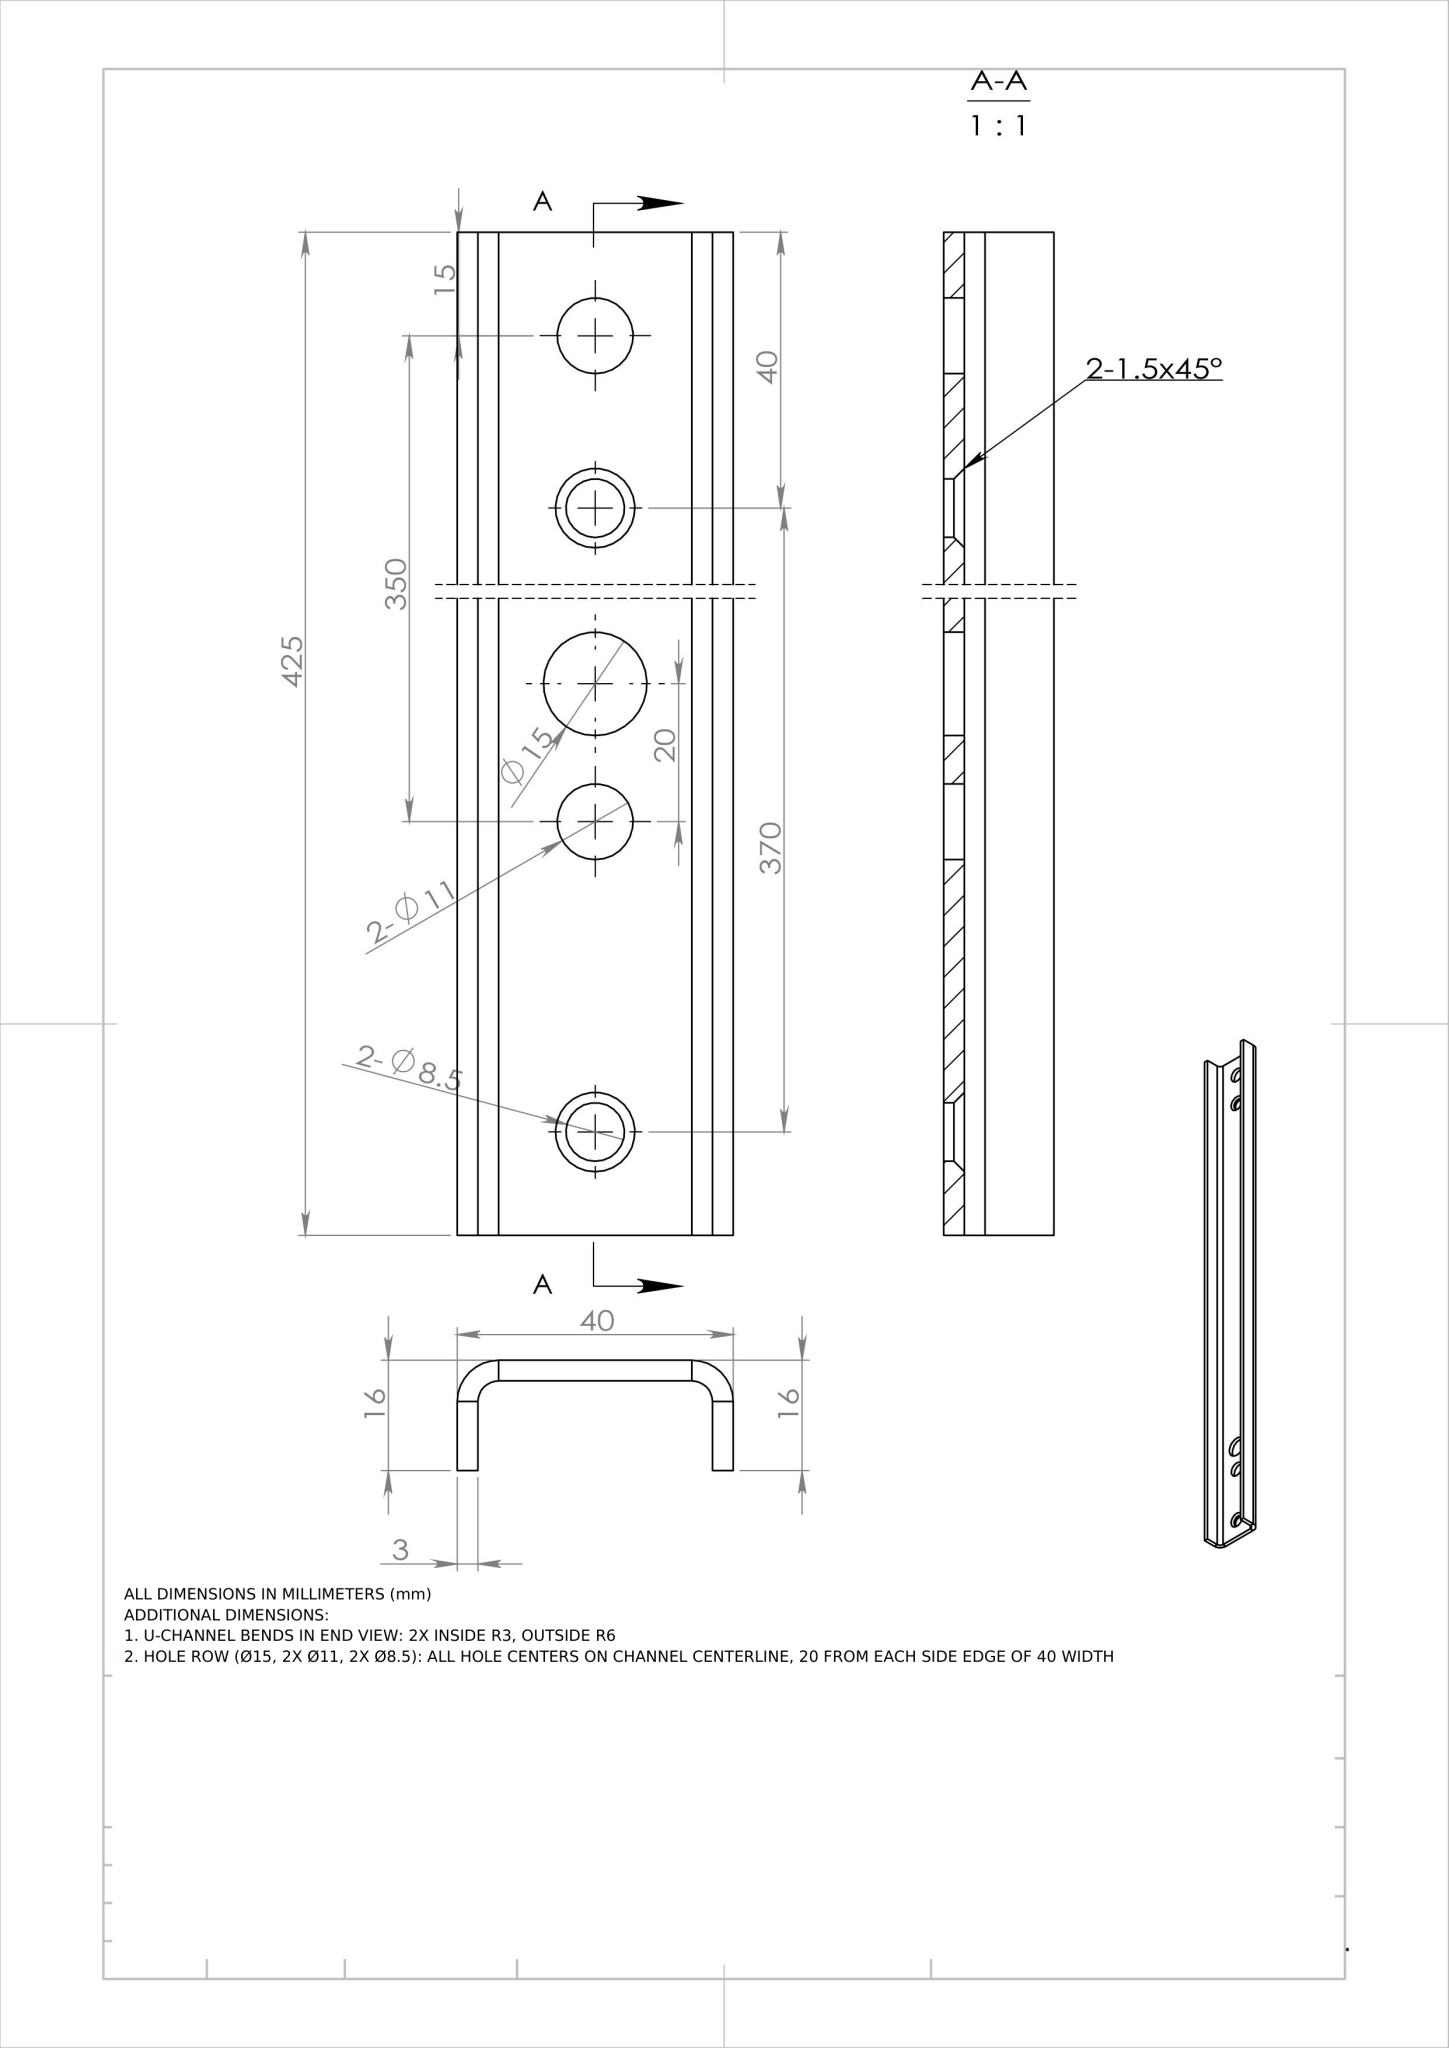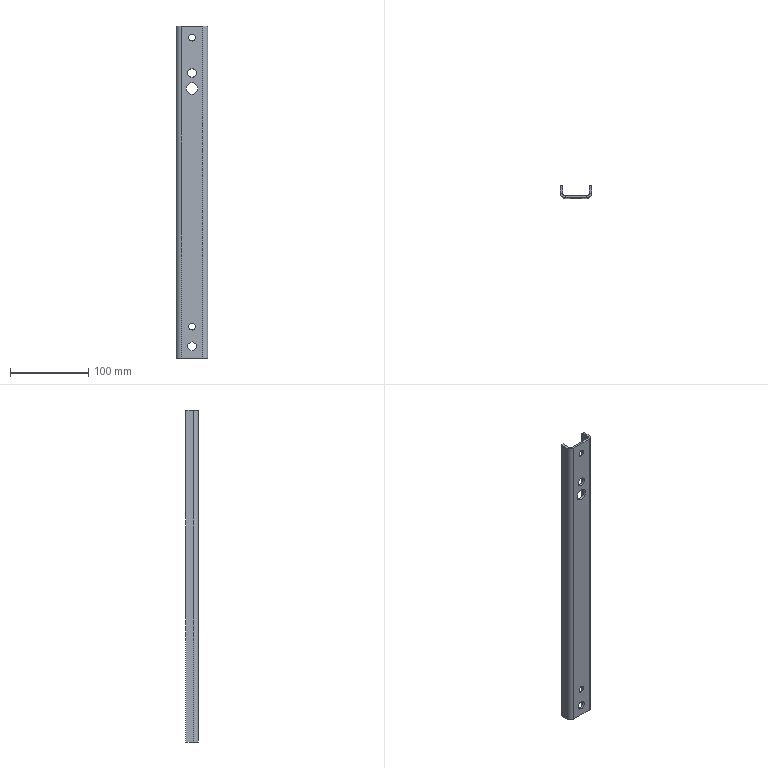Part | NX | mm | 1 solid | 36 faces | box 40 x 16 x 425 mm | volume 77717 mm3 | plane 18 | cylinder 14 | cone 4 | commonest cylinder face diameters 8.5 x4 11 x4 15 x2 12 x2 6 x2